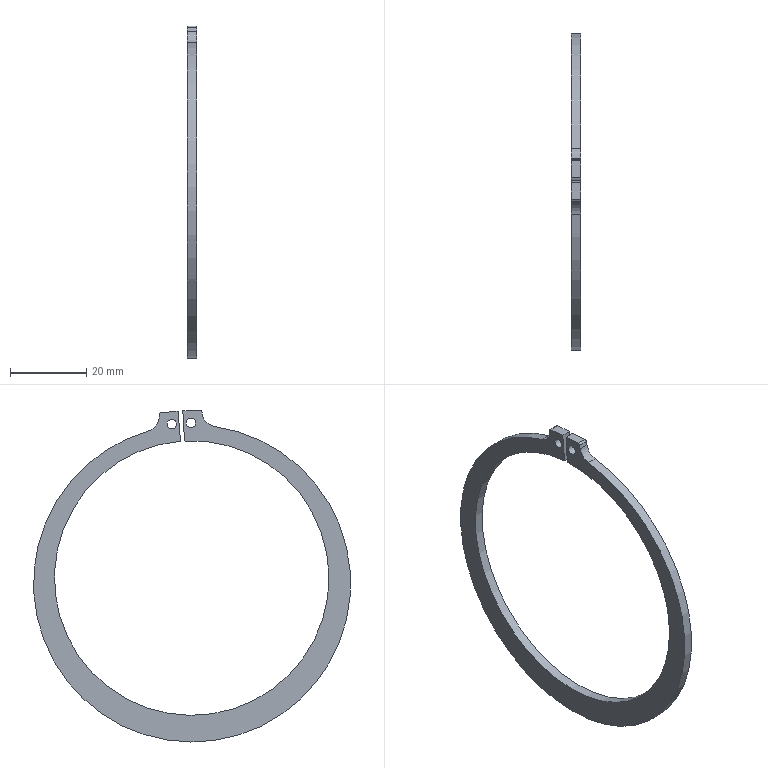Component | NX | SHAFT_CLIP | 1 solid | 16 faces | volume 3473 mm3 | cylinder 8 | plane 8 | commonest cylinder face diameters 1 x2 2.5 x2 7.4 x1 83.168 x1 7.401 x1 72 x1